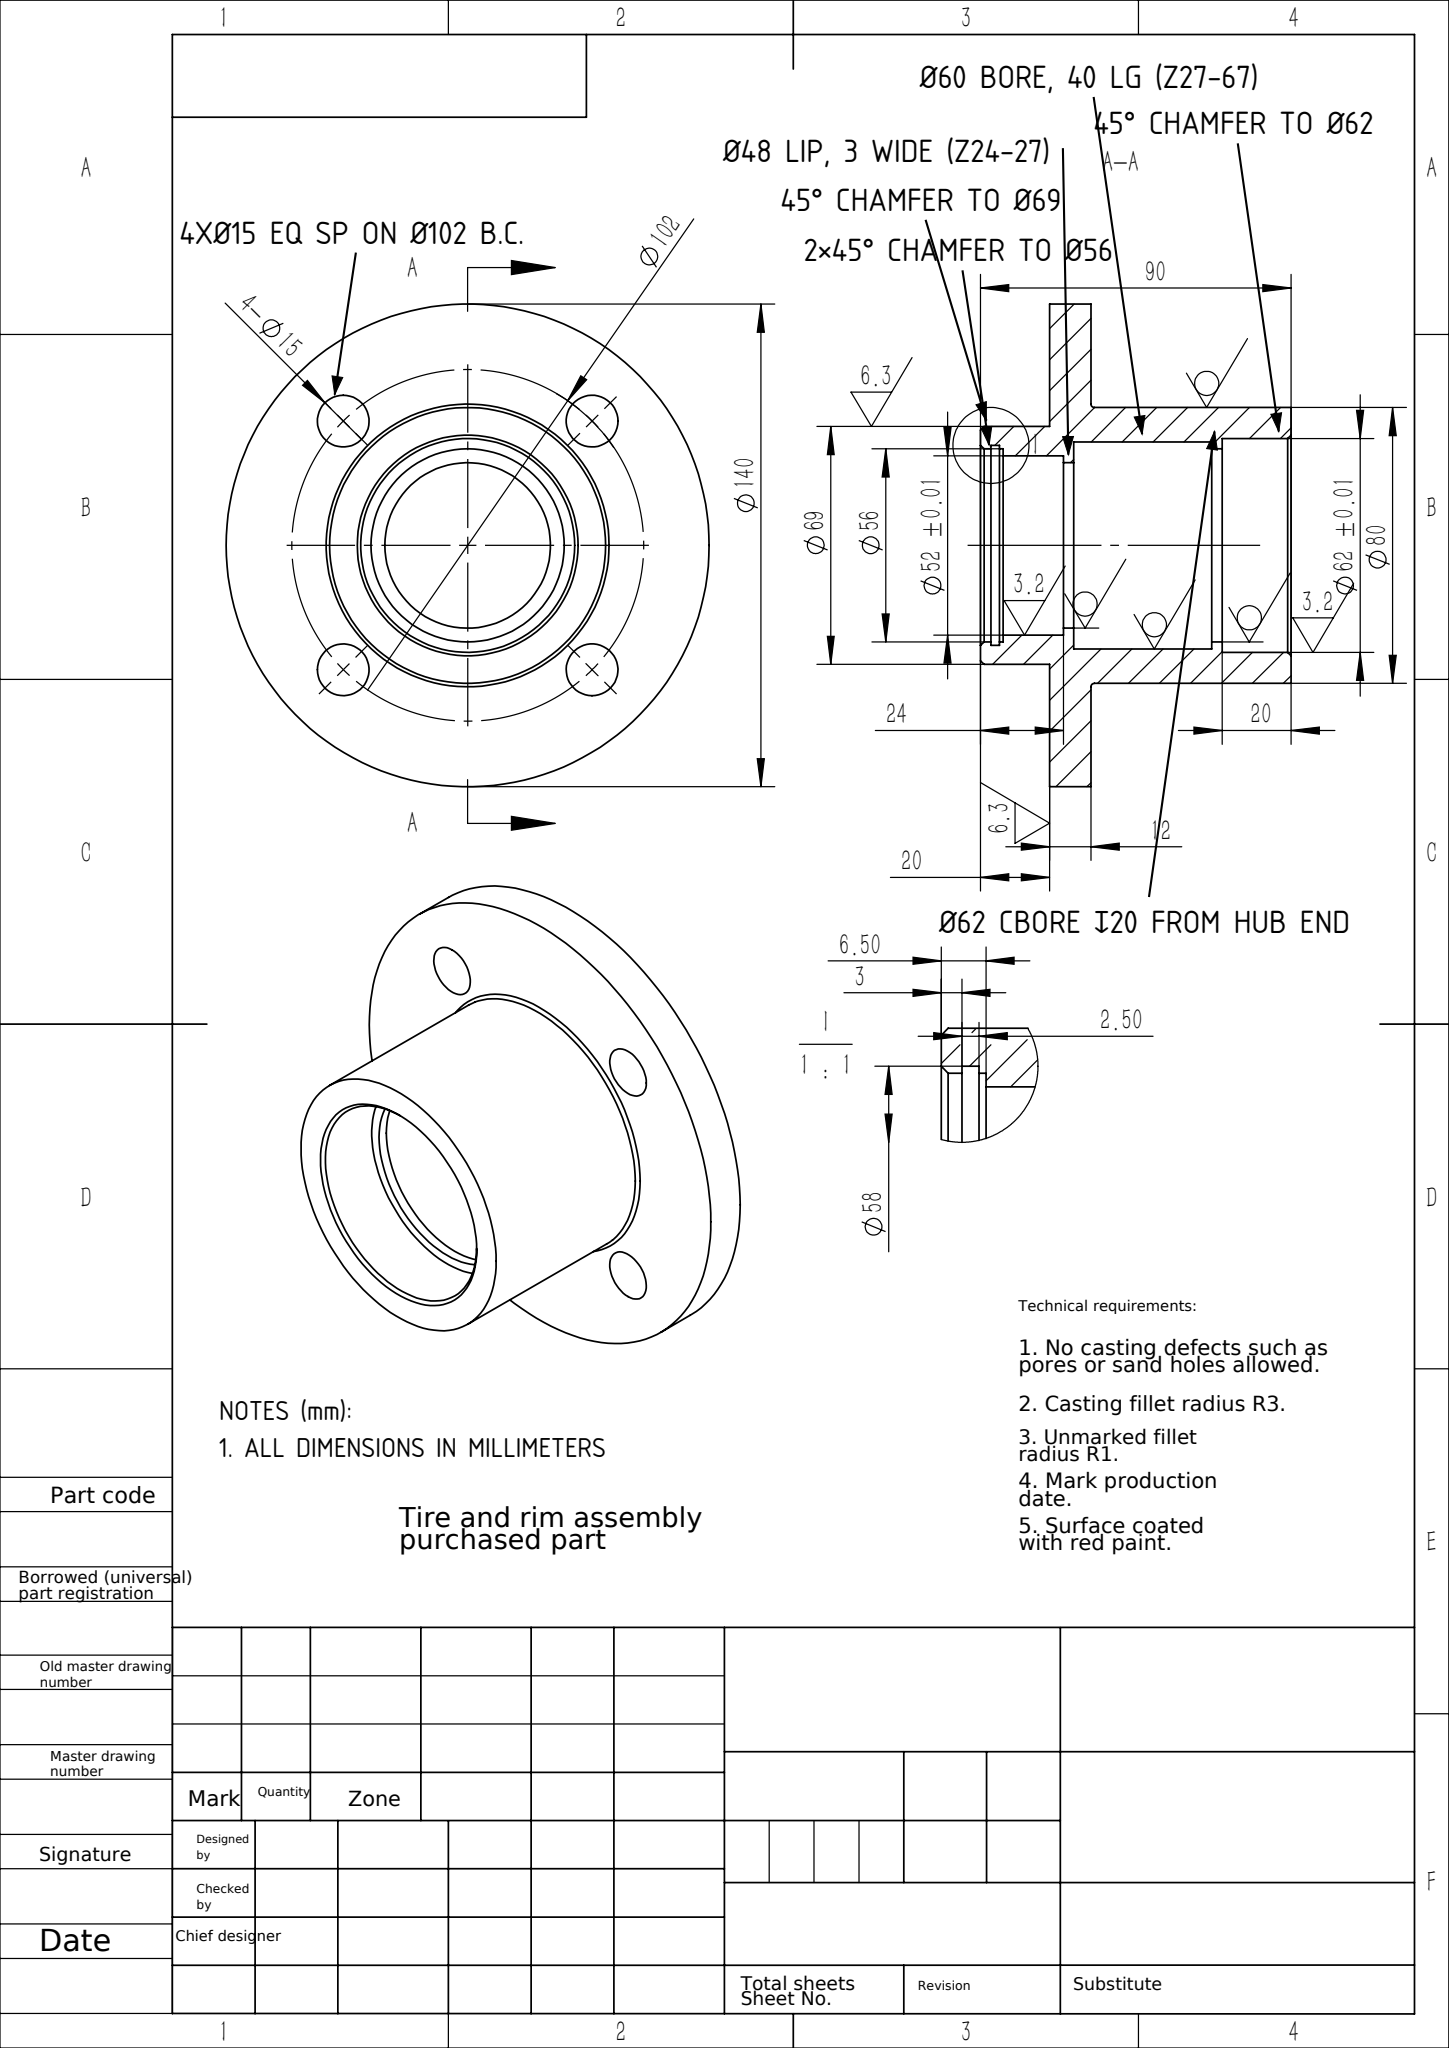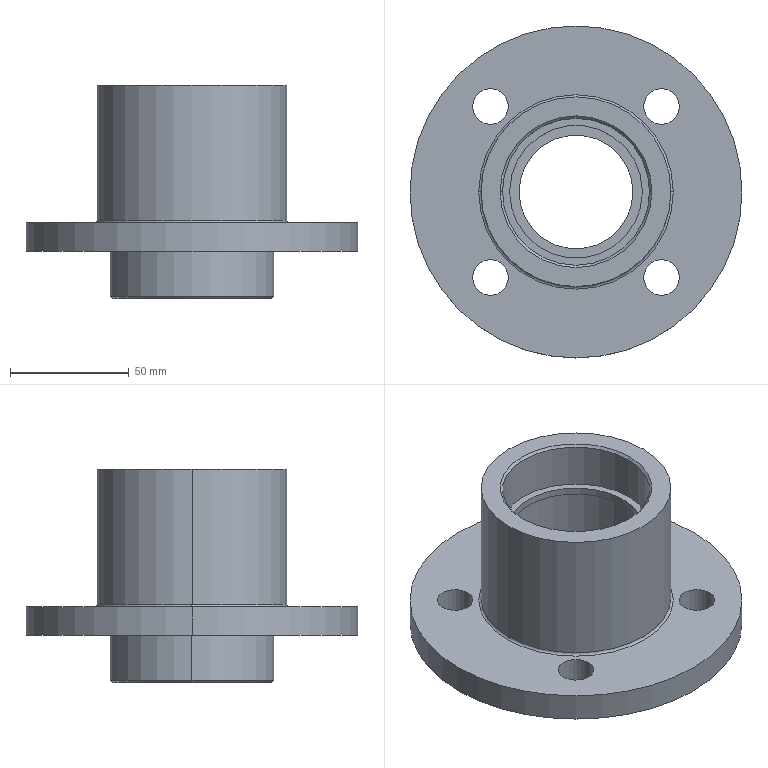Part | SolidWorks | mm | 1 solid | 49 faces | box 140 x 140 x 90 mm | volume 302409 mm3 | cylinder 30 | plane 11 | cone 6 | torus 2 | commonest cylinder face diameters 15 x8 56 x6 58 x2 60 x2 48 x2 52 x2 62 x2 80 x2
Drawing notes:
4X Ø15 THRU, EQUALLY SPACED 90° APART ON Ø102 BOLT CIRCLE, HOLE AXES AT 45° FROM FLANGE HORIZONTAL CENTERLINE; B.C. CONCENTRIC WITH PART AXIS (DATUM A) | from the solid: cylinders dia 15.0 axis z at (33.94,33.94), (33.94,106.06), (106.06,33.94), (106.06,106.06), length 12.0; part axis at (70,70) gives R51.0 = Ø102 B.C. with 90° spacing, 45° clocking
2 X 45° CHAMFER (90° INCLUDED) AT Ø52 BORE MOUTH, FLANGE END FACE (Z=0 DATUM B), BREAKING OUT TO Ø56 | from the solid: cones[included_angle 90.0, ref_dia 56.0]; cylinder dia 52.0 bore, length 17.5 from z=0 face
45° CHAMFER (90° INCLUDED) TO Ø62 AT BORE MOUTH ON HUB END FACE (Z=90 FROM DATUM B) | from the solid: cones[included_angle 90.0, ref_dia 62.0]; cylinder dia 62.0 length 19.0 at hub end
45° CHAMFER (90° INCLUDED) TO Ø69 AT Ø69 COUNTERBORE MOUTH, FLANGE END (Z=0 DATUM B) | from the solid: cones[included_angle 90.0, ref_dia 69.0]; cylinder dia 69.0 length 19.0
ALL DIMENSIONS IN MILLIMETERS | from the solid: STEP model units stated as mm
INTERNAL BORE Ø60 THRU-FEATURE, 40 LONG, FROM Z=27 TO Z=67 MEASURED FROM FLANGE END FACE (DATUM B, Z=0); COAXIAL WITH DATUM A | from the solid: cylinders: [60.0,"z",[70,70],40.0]; axis_planes z=27.0 and z=67.0
INTERNAL LIP Ø48, 3 WIDE, FROM Z=24 TO Z=27 FROM FLANGE END FACE (DATUM B, Z=0), BETWEEN Ø52 BORE AND Ø60 BORE; COAXIAL WITH DATUM A | from the solid: cylinders: [48.0,"z",[70,70],3.0]; axis_planes z=24.0 and z=27.0
STEP FROM Ø60 BORE TO Ø62±0.01 COUNTERBORE: Ø60 BORE ENDS AT Z=67 AND COUNTERBORE BOTTOM FACE AT Z=70 FROM FLANGE END FACE (DATUM B, Z=0), I.E. 3 APART; COUNTERBORE BOTTOM IS 20 FROM HUB END FACE (Z=90) | from the solid: axis_planes z=67.0 and z=70.0; cylinders [60.0,"z",40.0] and [62.0,"z",19.0]; bbox_xyz z=90
build123d program:
from build123d import *

# Parameters (mm, degrees)
SKETCH1_R           = 70
BOSS_EXTRUDE1_DEPTH = 12
SKETCH2_R           = 34.5
BOSS_EXTRUDE2_DEPTH = 20
SKETCH3_R           = 40
BOSS_EXTRUDE3_DEPTH = 58
SKETCH4_R           = 31
CUT_EXTRUDE1_DEPTH  = 20
SKETCH5_R           = 7.5
CUT_EXTRUDE2_DEPTH  = 25
CIRPATTERN1_COUNT   = 4
SKETCH7_R           = 28
CUT_EXTRUDE3_DEPTH  = 6.5
SKETCH8_R           = 26
CUT_EXTRUDE4_DEPTH  = 17.5
SKETCH9_R           = 24
CUT_EXTRUDE5_DEPTH  = 119.979
CHAMFER1_SIZE       = 1
FILLET3_R           = 1
CUT_EXTRUDE6_START  = -3
SKETCH11_R          = 30
CUT_EXTRUDE6_DEPTH  = 40
CUT_EXTRUDE7_START  = -5
SKETCH12_R          = 28
CUT_EXTRUDE7_DEPTH  = 5
SKETCH13_W          = 2
SKETCH13_H          = 2.5


with BuildPart() as part:
    # Sketch1 → Boss-Extrude1 (new body)
    with BuildSketch(Plane.XY):
        Circle(SKETCH1_R)
    extrude(amount=BOSS_EXTRUDE1_DEPTH)

    # Sketch2 → Boss-Extrude2 (add)
    with BuildSketch(Plane.XY):
        Circle(SKETCH2_R)
    extrude(amount=-BOSS_EXTRUDE2_DEPTH)

    # Sketch3 → Boss-Extrude3 (add)
    with BuildSketch(Plane.XY.offset(12)):
        with Locations(Location((0, 0, 0), (0, 0, 180))):
            Circle(SKETCH3_R)
    extrude(amount=BOSS_EXTRUDE3_DEPTH)

    # Sketch4 → Cut-Extrude1 (cut)
    with BuildSketch(Plane.XY.offset(70)):
        Circle(SKETCH4_R)
    extrude(amount=-CUT_EXTRUDE1_DEPTH, mode=Mode.SUBTRACT)

    # Sketch5 → Cut-Extrude2 (cut)
    with BuildSketch(Plane.XY.offset(12)):
        with Locations((36.062, 36.062)):
            Circle(SKETCH5_R)
    cut_extrude2 = extrude(amount=-CUT_EXTRUDE2_DEPTH, mode=Mode.SUBTRACT)

    # CirPattern1: Cut-Extrude2 ×4 about axis
    cirpattern1_axis = Axis((0, 0, 0), (0, 0, 1))
    for i in range(1, CIRPATTERN1_COUNT):
        add(cut_extrude2.rotate(cirpattern1_axis, i * 360 / CIRPATTERN1_COUNT), mode=Mode.SUBTRACT)

    # Sketch7 → Cut-Extrude3 (cut)
    with BuildSketch(Plane(origin=(0, 0, -20), x_dir=(-1, 0, 0), z_dir=(0, 0, -1))):
        Circle(SKETCH7_R)
    extrude(amount=-CUT_EXTRUDE3_DEPTH, mode=Mode.SUBTRACT)

    # Sketch8 → Cut-Extrude4 (cut)
    with BuildSketch(Plane(origin=(0, 0, -13.5), x_dir=(-1, 0, 0), z_dir=(0, 0, -1))):
        Circle(SKETCH8_R)
    extrude(amount=-CUT_EXTRUDE4_DEPTH, mode=Mode.SUBTRACT)

    # Sketch9 → Cut-Extrude5 (cut, through all)
    with BuildSketch(Plane(origin=(0, 0, 4), x_dir=(-1, 0, 0), z_dir=(0, 0, -1))):
        Circle(SKETCH9_R)
    extrude(amount=-CUT_EXTRUDE5_DEPTH, mode=Mode.SUBTRACT)

    # Chamfer1
    chamfer1_edges = [part.edges().sort_by_distance(p)[0] for p in [
        (-31, 0, 70),
        (28, 0, -20),
        (-34.5, 0, -20),
    ]]
    chamfer(chamfer1_edges, length=CHAMFER1_SIZE)

    # Fillet3
    fillet3_edges = [part.edges().sort_by_distance(p)[0] for p in [
        (40, 0, 12),
    ]]
    fillet(fillet3_edges, radius=FILLET3_R)

    # Sketch11 → Cut-Extrude6 (cut)
    with BuildSketch(Plane(origin=(0, 0, 4), x_dir=(-1, 0, 0), z_dir=(0, 0, -1)).offset(CUT_EXTRUDE6_START)):
        Circle(SKETCH11_R)
    extrude(amount=-CUT_EXTRUDE6_DEPTH, mode=Mode.SUBTRACT)

    # Sketch12 → Cut-Extrude7 (cut)
    with BuildSketch(Plane.XY.offset(50).offset(CUT_EXTRUDE7_START)):
        with Locations(Location((0, 0, 0), (0, 0, 180))):
            Circle(SKETCH12_R)
    extrude(amount=CUT_EXTRUDE7_DEPTH, mode=Mode.SUBTRACT)

    # Sketch13 → Cut-Revolve1 (revolve, cut)
    with BuildSketch(Plane(origin=(0, 0, 0), x_dir=(1, 0, 0), z_dir=(0, 1, 0)), mode=Mode.PRIVATE) as cut_revolve1_sk:
        with Locations((-28, 15.75)):
            Rectangle(SKETCH13_W, SKETCH13_H)
    revolve(cut_revolve1_sk.sketch.rotate(Axis((0, 0, 0), (0, 0, -1)), 180), axis=Axis((0, 0, 0), (0, 0, -1)), mode=Mode.SUBTRACT)


solid = part.part